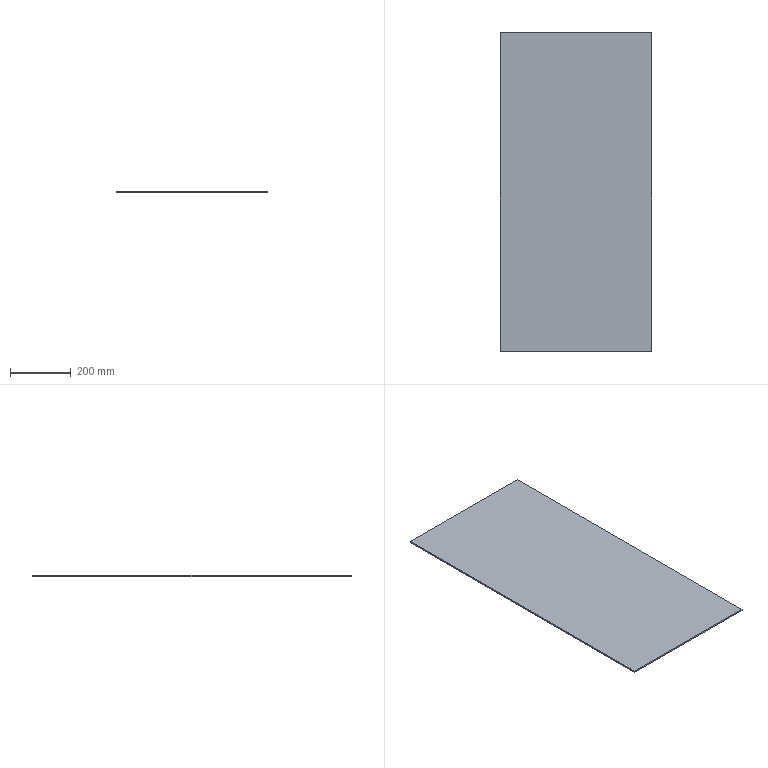Component | SolidWorks | BrownAcrylicPlate-5_BrownAcrylicPlate-4-1 | 1 solid | 6 faces | box 500 x 1050 x 5 mm | volume 2625000 mm3 | plane 6
build123d program:
from build123d import *

# Parameters (mm, degrees)
SKETCH1_W           = 500
SKETCH1_H           = 1050
BOSS_EXTRUDE1_DEPTH = 5


with BuildPart() as part:
    # Sketch1 → Boss-Extrude1 (new body)
    with BuildSketch(Plane(origin=(0, 0, 0), x_dir=(1, 0, 0), z_dir=(0, 1, 0))):
        Rectangle(SKETCH1_W, SKETCH1_H)
    extrude(amount=BOSS_EXTRUDE1_DEPTH)


solid = part.part

# Placed as in the assembly
solid = solid.moved(Location((360.5, 1525.65, -1336.5), (90, 0, 0)))
STEP:
#1=COLOUR_RGB('',0.7922,0.8196,0.9333);
#2=FILL_AREA_STYLE_COLOUR('',#1);
#3=FILL_AREA_STYLE('',(#2));
#4=SURFACE_STYLE_FILL_AREA(#3);
#5=SURFACE_SIDE_STYLE('',(#4));
#6=SURFACE_STYLE_USAGE(.BOTH.,#5);
#7=PRESENTATION_STYLE_ASSIGNMENT((#6));
#8=CARTESIAN_POINT('',(4.35,80.734,-52.618));
#9=VERTEX_POINT('',#8);
#10=CARTESIAN_POINT('',(24.035,80.734,-52.618));
#11=VERTEX_POINT('',#10);
#12=CARTESIAN_POINT('',(4.35,80.734,-52.618));
#13=DIRECTION('',(1.,-0.,-0.));
#14=VECTOR('',#13,39.37);
#15=LINE('',#12,#14);
#16=EDGE_CURVE('',#9,#11,#15,.T.);
#17=ORIENTED_EDGE('',*,*,#16,.F.);
#18=CARTESIAN_POINT('',(4.35,80.734,-52.421));
#19=VERTEX_POINT('',#18);
#20=CARTESIAN_POINT('',(4.35,80.734,-52.421));
#21=DIRECTION('',(-0.,-0.,-1.));
#22=VECTOR('',#21,39.37);
#23=LINE('',#20,#22);
#24=EDGE_CURVE('',#19,#9,#23,.T.);
#25=ORIENTED_EDGE('',*,*,#24,.F.);
#26=CARTESIAN_POINT('',(24.035,80.734,-52.421));
#27=VERTEX_POINT('',#26);
#28=CARTESIAN_POINT('',(4.35,80.734,-52.421));
#29=DIRECTION('',(1.,-0.,-0.));
#30=VECTOR('',#29,39.37);
#31=LINE('',#28,#30);
#32=EDGE_CURVE('',#19,#27,#31,.T.);
#33=ORIENTED_EDGE('',*,*,#32,.T.);
#34=CARTESIAN_POINT('',(24.035,80.734,-52.421));
#35=DIRECTION('',(-0.,-0.,-1.));
#36=VECTOR('',#35,39.37);
#37=LINE('',#34,#36);
#38=EDGE_CURVE('',#27,#11,#37,.T.);
#39=ORIENTED_EDGE('',*,*,#38,.T.);
#40=EDGE_LOOP('',(#17,#25,#33,#39));
#41=FACE_OUTER_BOUND('',#40,.T.);
#42=CARTESIAN_POINT('',(4.35,80.734,-52.421));
#43=DIRECTION('',(0.,1.,-0.));
#44=DIRECTION('',(-1.,0.,0.));
#45=AXIS2_PLACEMENT_3D('',#42,#43,#44);
#46=PLANE('',#45);
#47=ADVANCED_FACE('',(#41),#46,.T.);
#48=CARTESIAN_POINT('',(4.35,39.396,-52.618));
#49=VERTEX_POINT('',#48);
#50=CARTESIAN_POINT('',(4.35,80.734,-52.618));
#51=DIRECTION('',(-0.,-1.,0.));
#52=VECTOR('',#51,39.37);
#53=LINE('',#50,#52);
#54=EDGE_CURVE('',#9,#49,#53,.T.);
#55=ORIENTED_EDGE('',*,*,#54,.T.);
#56=CARTESIAN_POINT('',(4.35,39.396,-52.421));
#57=VERTEX_POINT('',#56);
#58=CARTESIAN_POINT('',(4.35,39.396,-52.421));
#59=DIRECTION('',(-0.,-0.,-1.));
#60=VECTOR('',#59,39.37);
#61=LINE('',#58,#60);
#62=EDGE_CURVE('',#57,#49,#61,.T.);
#63=ORIENTED_EDGE('',*,*,#62,.F.);
#64=CARTESIAN_POINT('',(4.35,80.734,-52.421));
#65=DIRECTION('',(-0.,-1.,0.));
#66=VECTOR('',#65,39.37);
#67=LINE('',#64,#66);
#68=EDGE_CURVE('',#19,#57,#67,.T.);
#69=ORIENTED_EDGE('',*,*,#68,.F.);
#70=ORIENTED_EDGE('',*,*,#24,.T.);
#71=EDGE_LOOP('',(#55,#63,#69,#70));
#72=FACE_OUTER_BOUND('',#71,.T.);
#73=CARTESIAN_POINT('',(4.35,80.734,-52.421));
#74=DIRECTION('',(1.,-0.,-0.));
#75=DIRECTION('',(0.,1.,-0.));
#76=AXIS2_PLACEMENT_3D('',#73,#74,#75);
#77=PLANE('',#76);
#78=ADVANCED_FACE('',(#72),#77,.F.);
#79=CARTESIAN_POINT('',(24.035,39.396,-52.618));
#80=VERTEX_POINT('',#79);
#81=CARTESIAN_POINT('',(4.35,39.396,-52.618));
#82=DIRECTION('',(1.,-0.,-0.));
#83=VECTOR('',#82,39.37);
#84=LINE('',#81,#83);
#85=EDGE_CURVE('',#49,#80,#84,.T.);
#86=ORIENTED_EDGE('',*,*,#85,.T.);
#87=CARTESIAN_POINT('',(24.035,39.396,-52.421));
#88=VERTEX_POINT('',#87);
#89=CARTESIAN_POINT('',(24.035,39.396,-52.421));
#90=DIRECTION('',(-0.,-0.,-1.));
#91=VECTOR('',#90,39.37);
#92=LINE('',#89,#91);
#93=EDGE_CURVE('',#88,#80,#92,.T.);
#94=ORIENTED_EDGE('',*,*,#93,.F.);
#95=CARTESIAN_POINT('',(4.35,39.396,-52.421));
#96=DIRECTION('',(1.,-0.,-0.));
#97=VECTOR('',#96,39.37);
#98=LINE('',#95,#97);
#99=EDGE_CURVE('',#57,#88,#98,.T.);
#100=ORIENTED_EDGE('',*,*,#99,.F.);
#101=ORIENTED_EDGE('',*,*,#62,.T.);
#102=EDGE_LOOP('',(#86,#94,#100,#101));
#103=FACE_OUTER_BOUND('',#102,.T.);
#104=CARTESIAN_POINT('',(4.35,39.396,-52.421));
#105=DIRECTION('',(0.,1.,-0.));
#106=DIRECTION('',(-1.,0.,0.));
#107=AXIS2_PLACEMENT_3D('',#104,#105,#106);
#108=PLANE('',#107);
#109=ADVANCED_FACE('',(#103),#108,.F.);
#110=CARTESIAN_POINT('',(24.035,80.734,-52.618));
#111=DIRECTION('',(-0.,-1.,0.));
#112=VECTOR('',#111,39.37);
#113=LINE('',#110,#112);
#114=EDGE_CURVE('',#11,#80,#113,.T.);
#115=ORIENTED_EDGE('',*,*,#114,.F.);
#116=ORIENTED_EDGE('',*,*,#38,.F.);
#117=CARTESIAN_POINT('',(24.035,80.734,-52.421));
#118=DIRECTION('',(-0.,-1.,0.));
#119=VECTOR('',#118,39.37);
#120=LINE('',#117,#119);
#121=EDGE_CURVE('',#27,#88,#120,.T.);
#122=ORIENTED_EDGE('',*,*,#121,.T.);
#123=ORIENTED_EDGE('',*,*,#93,.T.);
#124=EDGE_LOOP('',(#115,#116,#122,#123));
#125=FACE_OUTER_BOUND('',#124,.T.);
#126=CARTESIAN_POINT('',(24.035,80.734,-52.421));
#127=DIRECTION('',(1.,-0.,-0.));
#128=DIRECTION('',(0.,1.,-0.));
#129=AXIS2_PLACEMENT_3D('',#126,#127,#128);
#130=PLANE('',#129);
#131=ADVANCED_FACE('',(#125),#130,.T.);
#132=ORIENTED_EDGE('',*,*,#32,.F.);
#133=ORIENTED_EDGE('',*,*,#68,.T.);
#134=ORIENTED_EDGE('',*,*,#99,.T.);
#135=ORIENTED_EDGE('',*,*,#121,.F.);
#136=EDGE_LOOP('',(#132,#133,#134,#135));
#137=FACE_OUTER_BOUND('',#136,.T.);
#138=CARTESIAN_POINT('',(14.193,60.065,-52.421));
#139=DIRECTION('',(-0.,-0.,-1.));
#140=DIRECTION('',(0.,1.,-0.));
#141=AXIS2_PLACEMENT_3D('',#138,#139,#140);
#142=PLANE('',#141);
#143=ADVANCED_FACE('',(#137),#142,.F.);
#144=ORIENTED_EDGE('',*,*,#16,.T.);
#145=ORIENTED_EDGE('',*,*,#114,.T.);
#146=ORIENTED_EDGE('',*,*,#85,.F.);
#147=ORIENTED_EDGE('',*,*,#54,.F.);
#148=EDGE_LOOP('',(#144,#145,#146,#147));
#149=FACE_OUTER_BOUND('',#148,.T.);
#150=CARTESIAN_POINT('',(14.193,60.065,-52.618));
#151=DIRECTION('',(-0.,-0.,-1.));
#152=DIRECTION('',(0.,1.,-0.));
#153=AXIS2_PLACEMENT_3D('',#150,#151,#152);
#154=PLANE('',#153);
#155=ADVANCED_FACE('',(#149),#154,.T.);
#156=CLOSED_SHELL('',(#47,#78,#109,#131,#143,#155));
#157=MANIFOLD_SOLID_BREP('',#156);
#158=STYLED_ITEM('',(#7),#157);
#159=PRESENTATION_LAYER_ASSIGNMENT('','',(#158));
#160=CARTESIAN_POINT('',(0.,0.,0.));
#161=DIRECTION('',(0.,0.,1.));
#162=DIRECTION('',(1.,0.,0.));
#163=AXIS2_PLACEMENT_3D('',#160,#161,#162);
#164=(LENGTH_UNIT()NAMED_UNIT(*)SI_UNIT($,.METRE.));
#165=LENGTH_MEASURE_WITH_UNIT(LENGTH_MEASURE(0.0254),#164);
#166=DIMENSIONAL_EXPONENTS(1.,0.,0.,0.,0.,0.,0.);
#167=(CONVERSION_BASED_UNIT('',#165)LENGTH_UNIT()NAMED_UNIT(#166));
#168=UNCERTAINTY_MEASURE_WITH_UNIT(LENGTH_MEASURE(0.00001),#167,'','');
#169=(NAMED_UNIT(*)PLANE_ANGLE_UNIT()SI_UNIT($,.RADIAN.));
#170=(NAMED_UNIT(*)SI_UNIT($,.STERADIAN.)SOLID_ANGLE_UNIT());
#171=(GEOMETRIC_REPRESENTATION_CONTEXT(3)GLOBAL_UNCERTAINTY_ASSIGNED_CONTEXT((#168))GLOBAL_UNIT_ASSIGNED_CONTEXT((#167,#169,#170))REPRESENTATION_CONTEXT('',''));
#172=ADVANCED_BREP_SHAPE_REPRESENTATION('',(#157,#163),#171);
#173=(LENGTH_UNIT()NAMED_UNIT(*)SI_UNIT($,.METRE.));
#174=LENGTH_MEASURE_WITH_UNIT(LENGTH_MEASURE(0.0254),#173);
#175=DIMENSIONAL_EXPONENTS(1.,0.,0.,0.,0.,0.,0.);
#176=(CONVERSION_BASED_UNIT('',#174)LENGTH_UNIT()NAMED_UNIT(#175));
#177=UNCERTAINTY_MEASURE_WITH_UNIT(LENGTH_MEASURE(0.00001),#176,'','');
#178=(NAMED_UNIT(*)PLANE_ANGLE_UNIT()SI_UNIT($,.RADIAN.));
#179=(NAMED_UNIT(*)SI_UNIT($,.STERADIAN.)SOLID_ANGLE_UNIT());
#180=(GEOMETRIC_REPRESENTATION_CONTEXT(3)GLOBAL_UNCERTAINTY_ASSIGNED_CONTEXT((#177))GLOBAL_UNIT_ASSIGNED_CONTEXT((#176,#178,#179))REPRESENTATION_CONTEXT('',''));
#181=MECHANICAL_DESIGN_GEOMETRIC_PRESENTATION_REPRESENTATION('',(#158),#180);